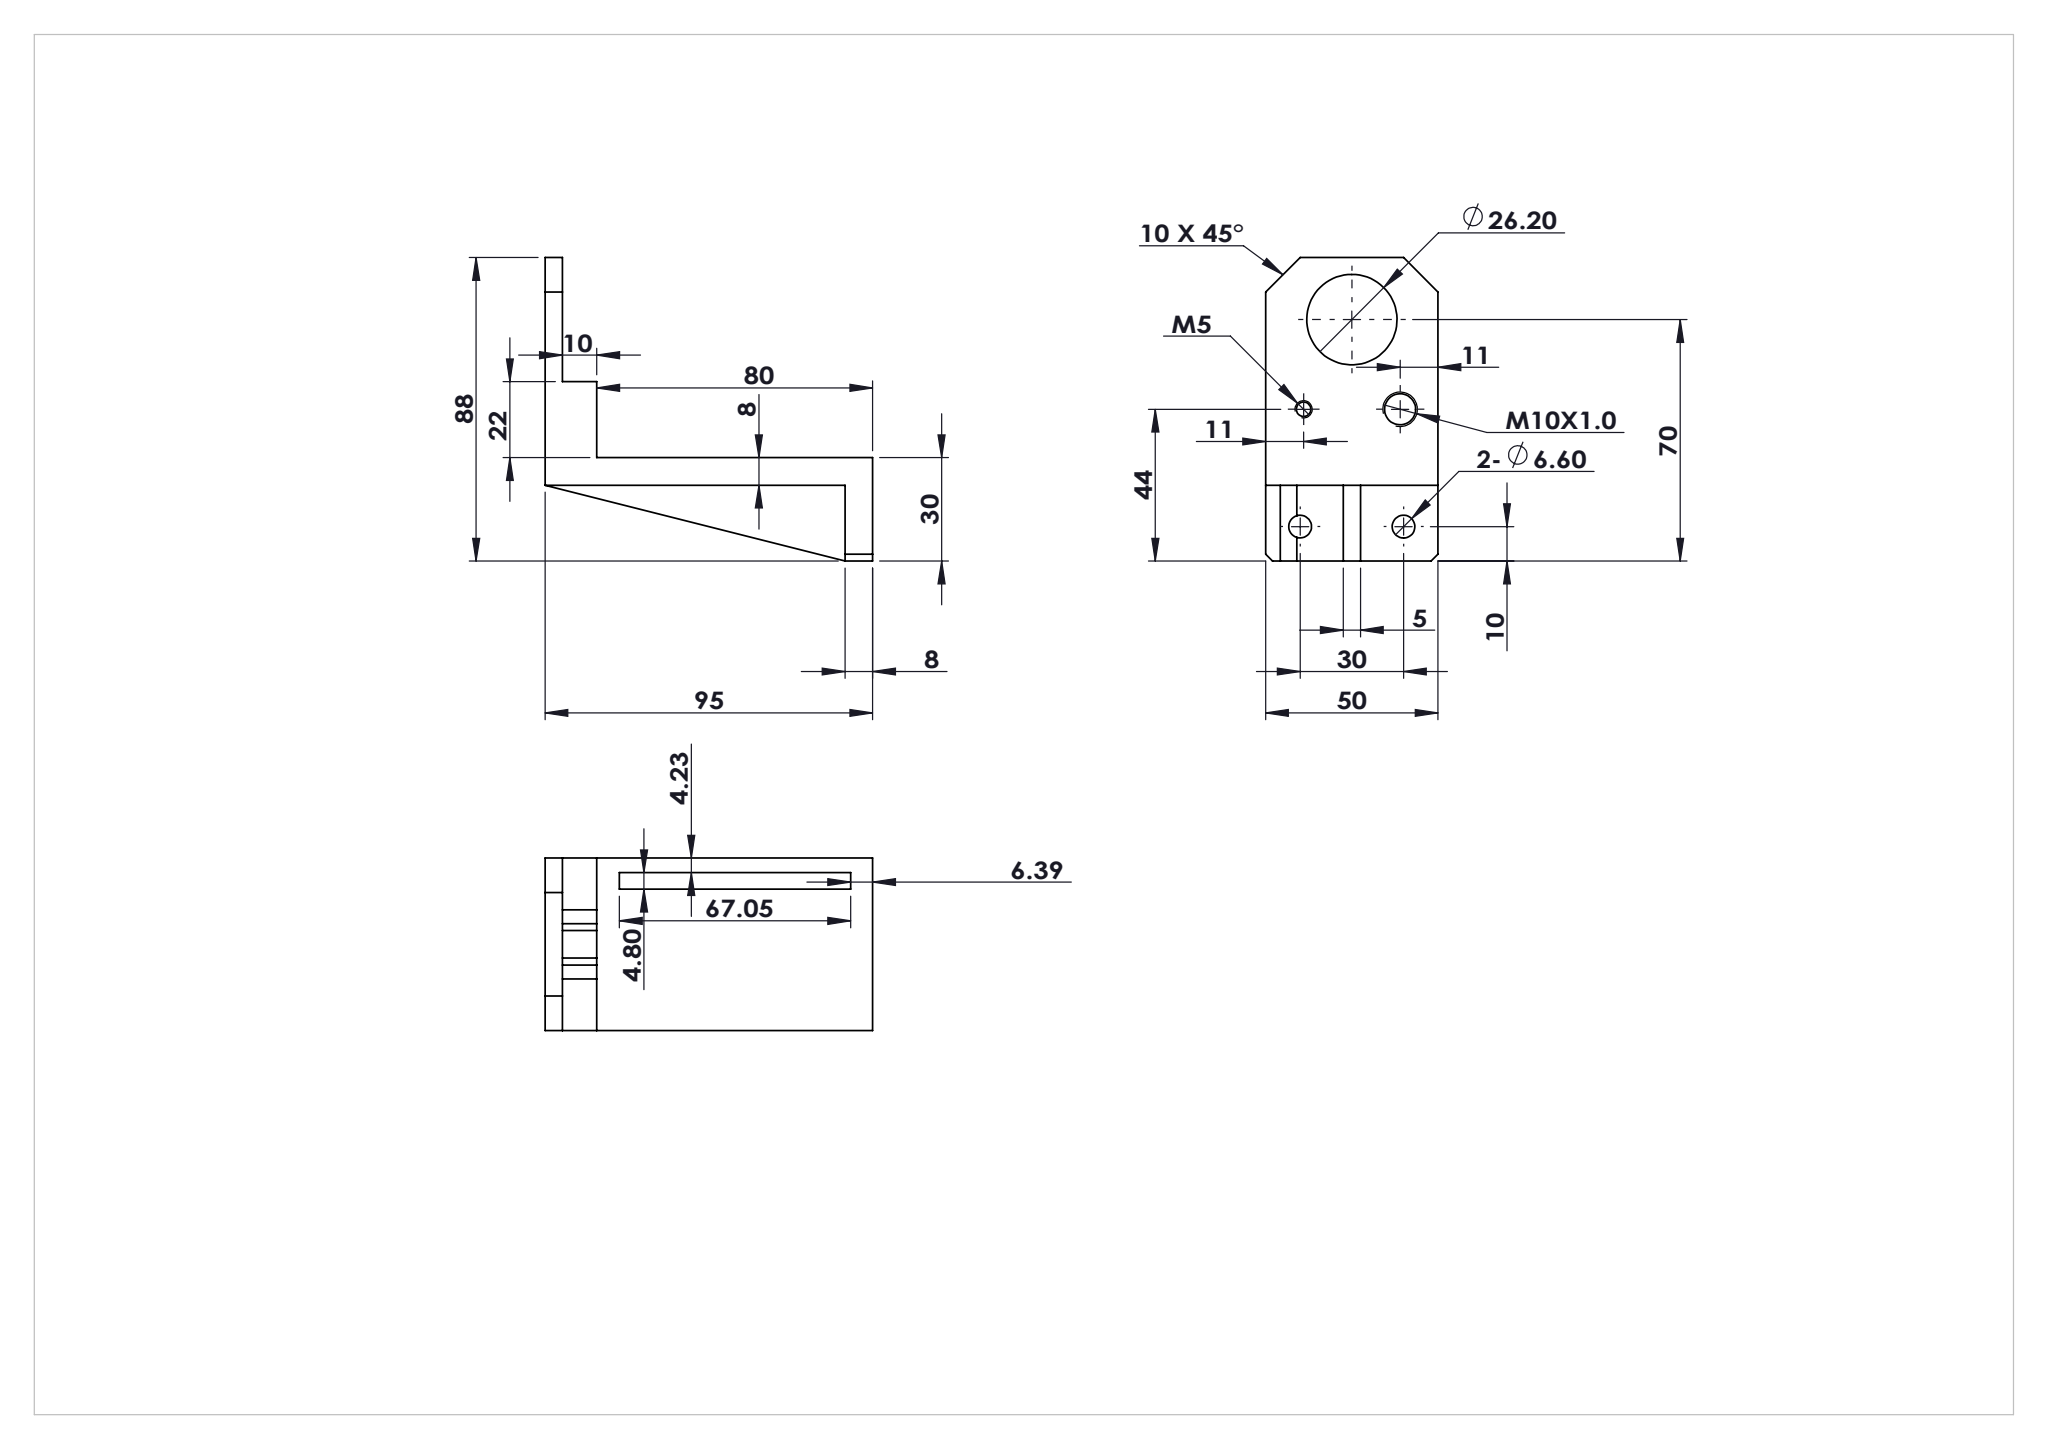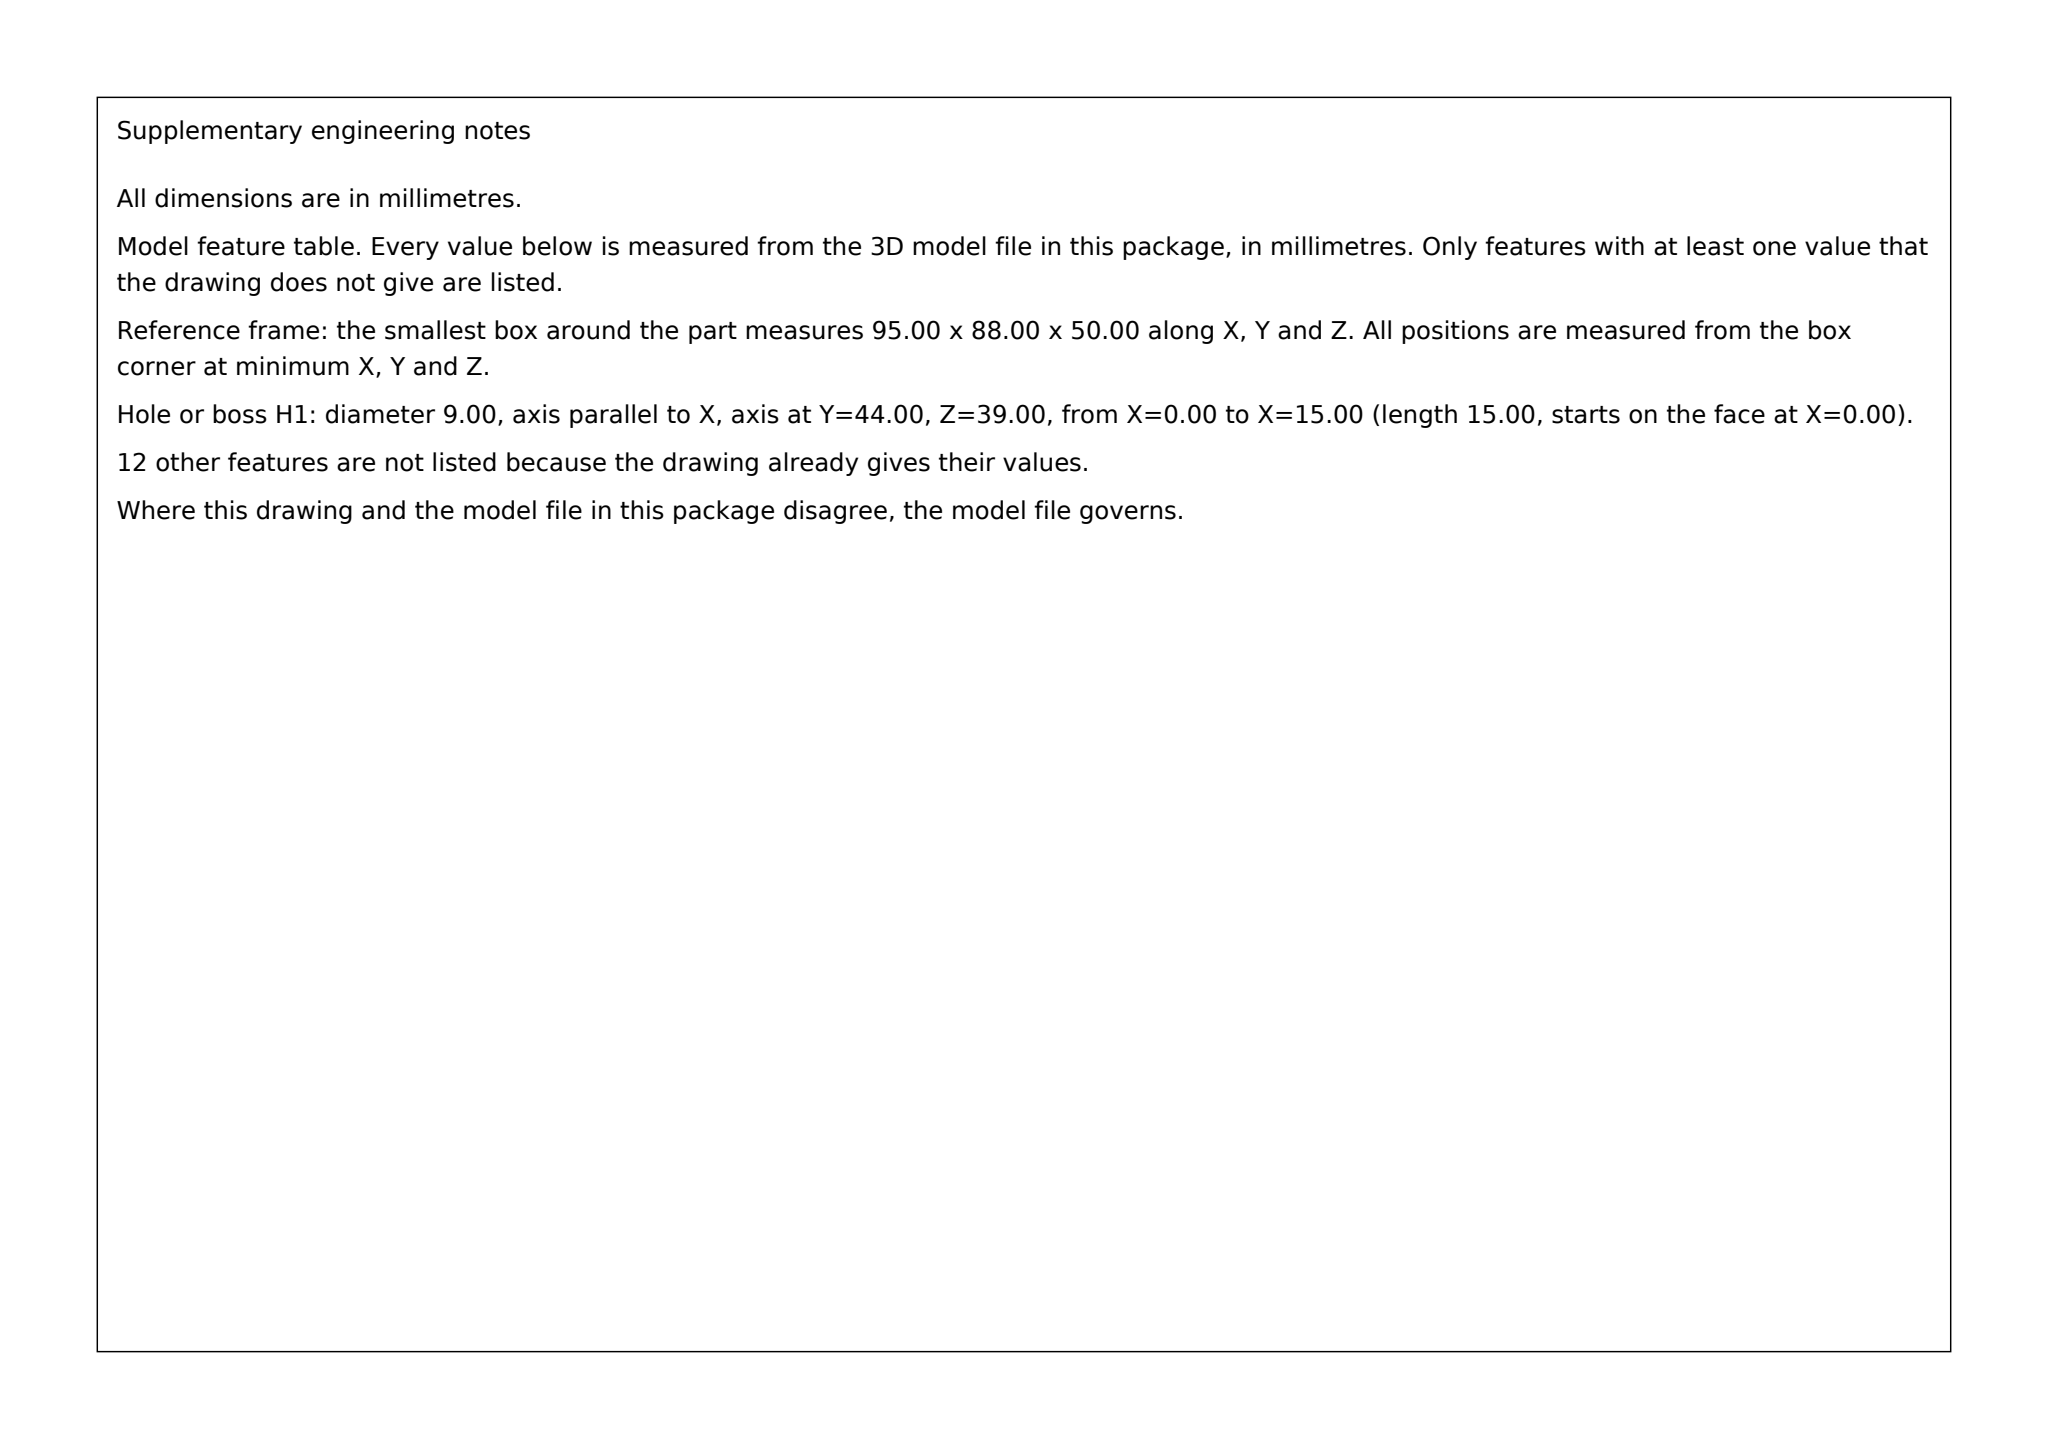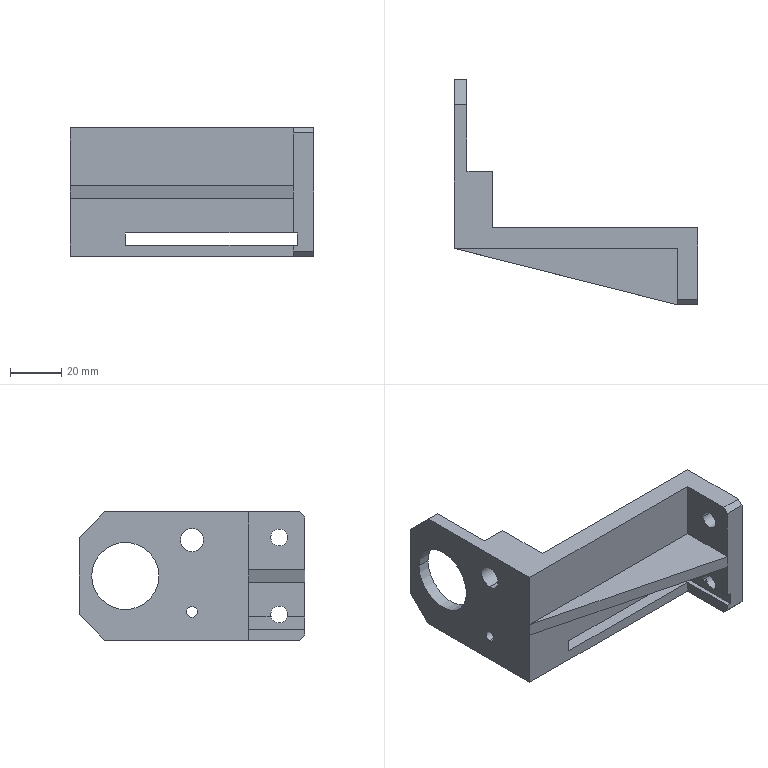Part | SolidWorks | mm | 1 solid | 45 faces | box 95 x 88 x 50 mm | volume 68321 mm3 | plane 33 | cylinder 12 | commonest cylinder face diameters 6.6 x4 4.2 x2 9 x2 26.2 x2 4 x2
build123d program:
from build123d import *

# Parameters (mm, degrees)
BOSS_EXTRUDE1_DEPTH    = 25
SKETCH2_R              = 13.1
CUT_EXTRUDE1_DEPTH     = 110.95
BOSS_EXTRUDE2_DEPTH    = 2.5
SKETCH11_W             = 50
SKETCH11_H             = 22
BOSS_EXTRUDE5_DEPTH    = 10
M10X1_0_TAPPED_HOLE2_D = 9
M5_TAPPED_HOLE1_D      = 4.2
CHAMFER1_SIZE          = 10
SKETCH18_R             = 3.3
CUT_EXTRUDE2_DEPTH     = 108.508
CHAMFER2_SIZE          = 2
SKETCH19_W             = 12
SKETCH19_H             = 8
CUT_EXTRUDE3_DEPTH     = 10
CHAMFER3_SIZE          = 4
FILLET1_R              = 2
SKETCH20_W             = 67.05
SKETCH20_H             = 4.795
CUT_EXTRUDE4_DEPTH     = 47


with BuildPart() as part:
    # Sketch1 → Boss-Extrude1 (new, symmetric)
    with BuildSketch(Plane.XY):
        Polygon((-90, 58), (-90, 0), (0, 0), (0, -30), (-8, -30), (-8, -8), (-95, -8), (-95, 58), align=None)
    extrude(amount=BOSS_EXTRUDE1_DEPTH, both=True)

    # Sketch2 → Cut-Extrude1 (cut, through all)
    with BuildSketch(Plane(origin=(-90, 0, 0), x_dir=(0, 0, -1), z_dir=(1, 0, 0))):
        with Locations(Location((0, 40, 0), (0, 0, 90))):
            Circle(SKETCH2_R)
    extrude(amount=-CUT_EXTRUDE1_DEPTH, mode=Mode.SUBTRACT)

    # Sketch3 → Boss-Extrude2 (add, symmetric)
    with BuildSketch(Plane.XY):
        Polygon((-8, -30), (-95, -8), (-8, -8), align=None)
    extrude(amount=BOSS_EXTRUDE2_DEPTH, both=True)

    # Sketch11 → Boss-Extrude5 (add)
    with BuildSketch(Plane(origin=(-90, 0, 0), x_dir=(0, 0, -1), z_dir=(1, 0, 0))):
        with Locations((0, 11)):
            Rectangle(SKETCH11_W, SKETCH11_H)
    extrude(amount=BOSS_EXTRUDE5_DEPTH)

    # M10x1.0 Tapped Hole2 (through all)
    with Locations(Plane.ZY.offset(95)):
        with Locations((14, 14)):
            Hole(M10X1_0_TAPPED_HOLE2_D / 2)

    # M5 Tapped Hole1 (through all)
    with Locations(Plane.ZY.offset(95)):
        with Locations((-14, 14)):
            Hole(M5_TAPPED_HOLE1_D / 2)

    # Chamfer1
    chamfer1_edges = [part.edges().sort_by_distance(p)[0] for p in [
        (-92.5, 58, -25),
        (-92.5, 58, 25),
    ]]
    chamfer(chamfer1_edges, length=CHAMFER1_SIZE)

    # Sketch18 → Cut-Extrude2 (cut, through all)
    with BuildSketch(Plane.ZY.offset(8)):
        with Locations(Location((15, -20, 0), (0, 0, 270))):
            Circle(SKETCH18_R)
        with Locations(Location((-15, -20, 0), (0, 0, 90))):
            Circle(SKETCH18_R)
    extrude(amount=-CUT_EXTRUDE2_DEPTH, mode=Mode.SUBTRACT)

    # Chamfer2
    chamfer2_edges = [part.edges().sort_by_distance(p)[0] for p in [
        (-4, -30, 25),
        (-4, -30, -25),
    ]]
    chamfer(chamfer2_edges, length=CHAMFER2_SIZE)

    # Sketch19 → Cut-Extrude3 (cut)
    with BuildSketch(Plane(origin=(-80, 0, 0), x_dir=(0, 0, -1), z_dir=(1, 0, 0))):
        with Locations((0, 18)):
            Rectangle(SKETCH19_W, SKETCH19_H)
    extrude(amount=-CUT_EXTRUDE3_DEPTH, mode=Mode.SUBTRACT)

    # Chamfer3
    chamfer3_edges = [part.edges().sort_by_distance(p)[0] for p in [
        (-85, 22, -6),
        (-85, 22, 6),
    ]]
    chamfer(chamfer3_edges, length=CHAMFER3_SIZE)

    # Fillet1
    fillet1_edges = [part.edges().sort_by_distance(p)[0] for p in [
        (-85, 14, -6),
        (-85, 14, 6),
    ]]
    fillet(fillet1_edges, radius=FILLET1_R)

    # Sketch20 → Cut-Extrude4 (cut)
    with BuildSketch(Plane(origin=(0, 0, 0), x_dir=(1, 0, 0), z_dir=(0, 1, 0))):
        with Locations((-39.919, 18.368)):
            Rectangle(SKETCH20_W, SKETCH20_H)
    extrude(amount=-CUT_EXTRUDE4_DEPTH, mode=Mode.SUBTRACT)


solid = part.part